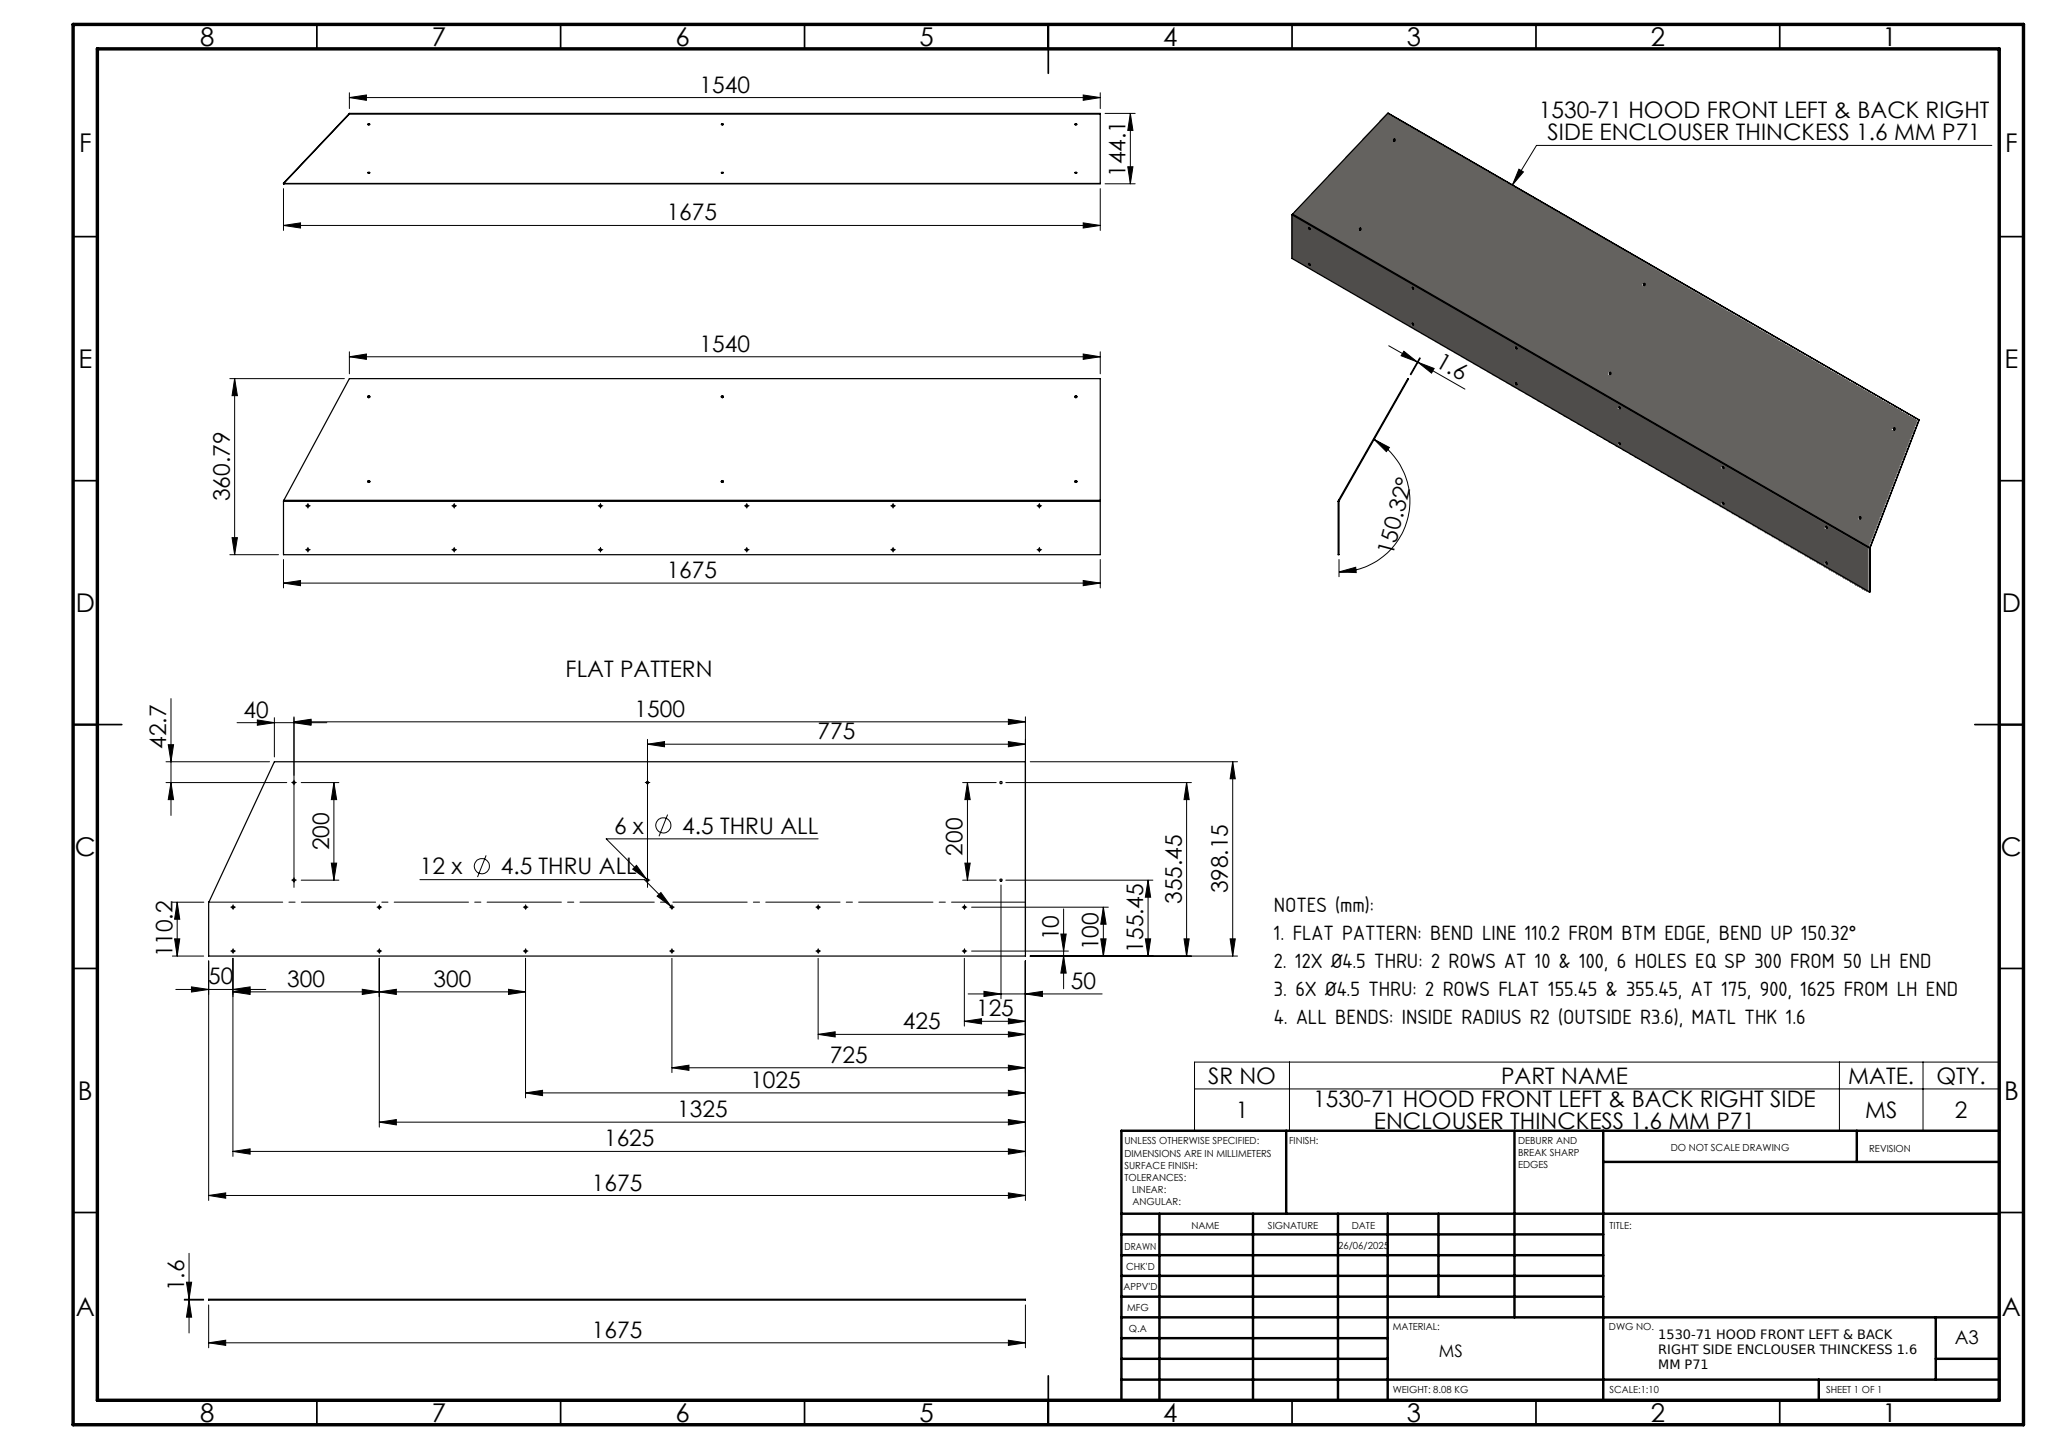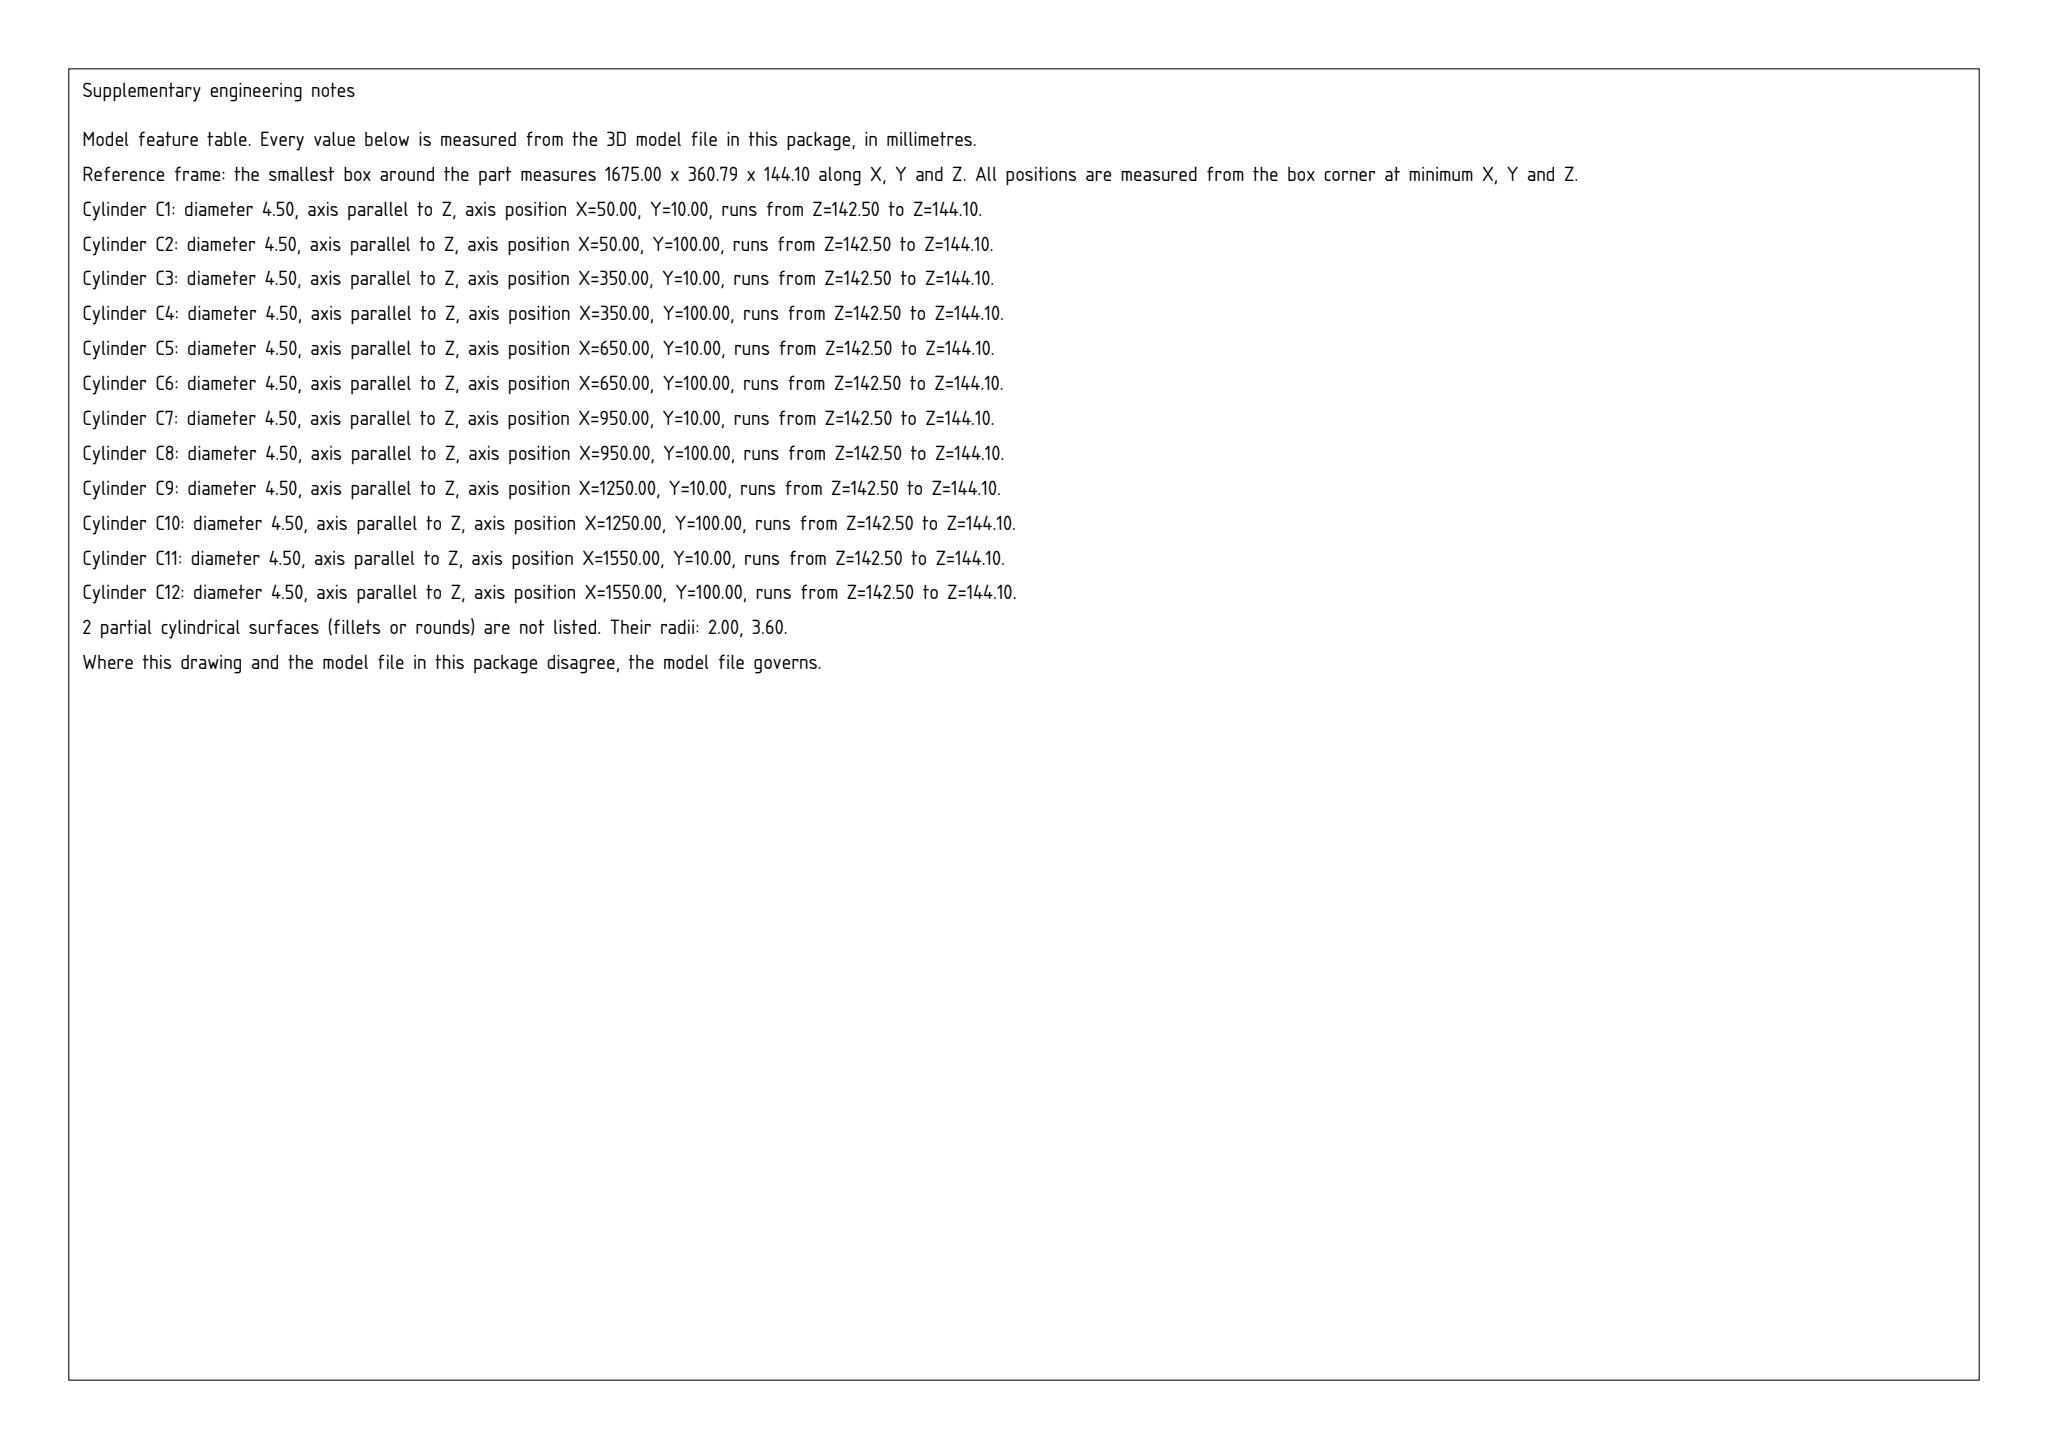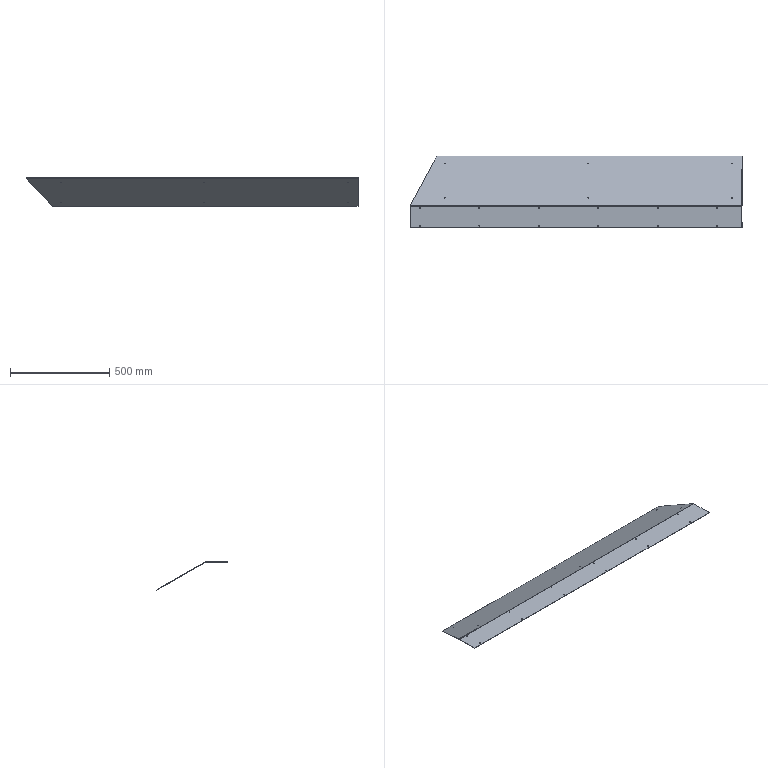Part | SolidWorks | mm | 1 solid | 51 faces | box 1675 x 360.79 x 144.1 mm | volume 1035411 mm3 | cylinder 38 | plane 12 | spline 1 | commonest cylinder face diameters 4.5 x36 4 x1 7.2 x1
Drawing notes:
FLAT PATTERN: BEND LINE 110.2 FROM BTM EDGE, BEND UP 150.32° | from the solid: Lower holes y=10/100 L=1.6 vs upper y=149.94/323.7 L=3.62 inclined; bbox Y=360.792
12X Ø4.5 THRU: 2 ROWS AT 10 & 100, 6 HOLES EQ SP 300 FROM 50 LH END | from the solid: Ø4.5 z-holes x=50,350,650,950,1250,1550 at y=10 and y=100 (12 total, L=1.6)
6X Ø4.5 THRU: 2 ROWS FLAT 155.45 & 355.45, AT 175, 900, 1625 FROM LH END | from the solid: Ø4.5 z-holes x=175,900,1625 at y=149.94 and y=323.7 (6 total, L=3.62); = 1500/775/50 from RH end
ALL BENDS: INSIDE RADIUS R2 (OUTSIDE R3.6), MATL THK 1.6 | from the solid: cylinders dia 4.0 and 7.2 about x-axis at y=109.47, z=140.5, len 1675 -> inner R2.0 / outer R3.6 bend along 1675 bend line